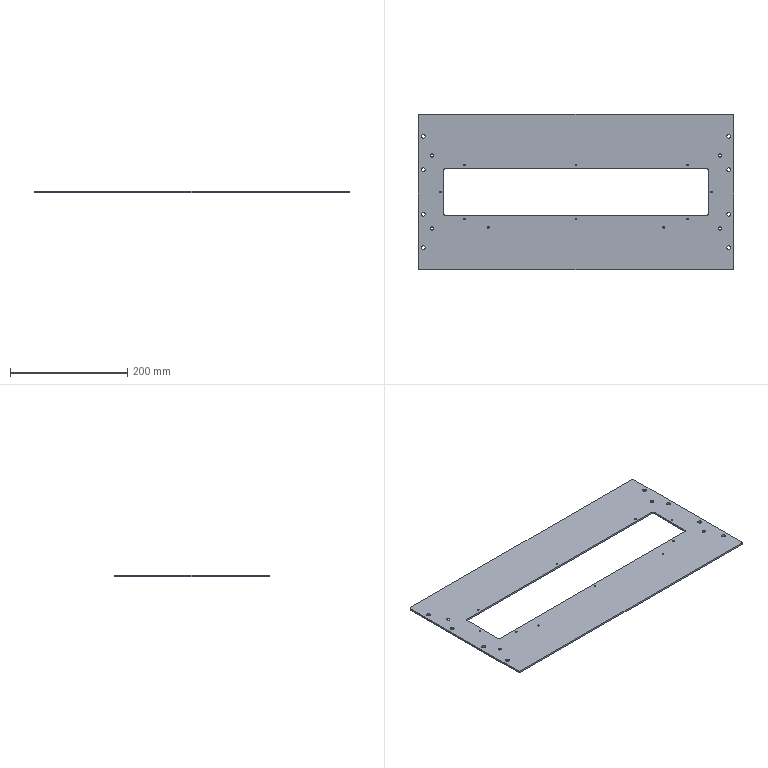CAM job | Mastercam | mm | 6 operations | part box 540 x 266 x 3
1. Contour (Ramp) | 9 - 10 平铣刀
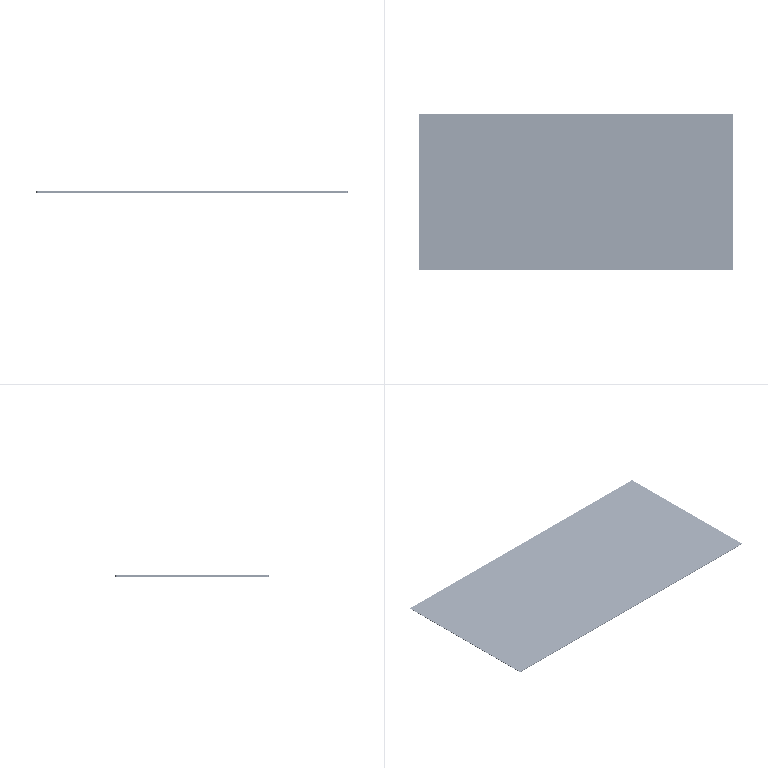2. Contour (2D) | 10 - 10 平铣刀
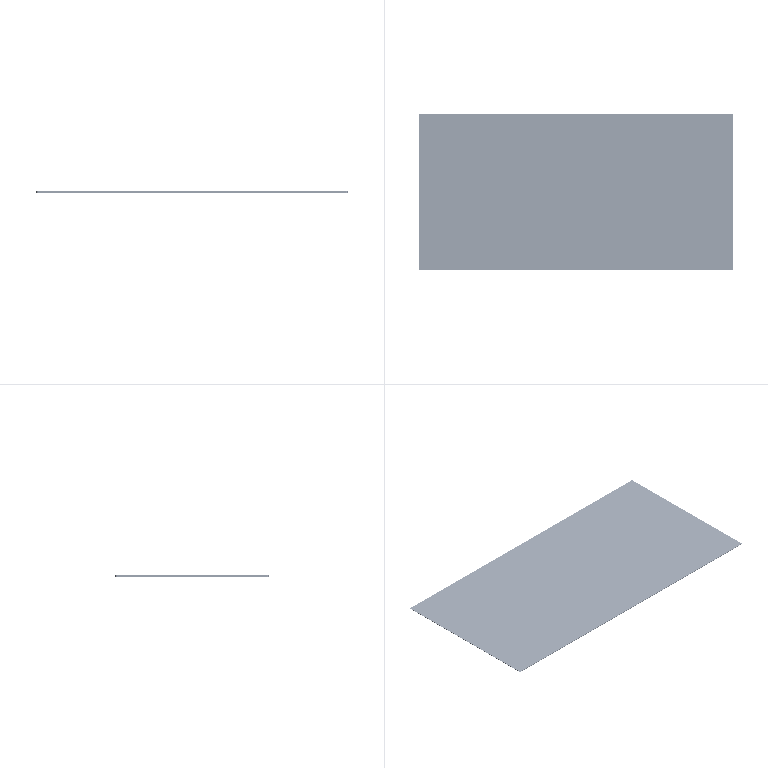3. Contour (Ramp) | 4 - 4 平铣刀
4. Drill/Counterbore | 7 - 4 倒角刀
5. Contour (2D chamfer) | 7 - 4 倒角刀
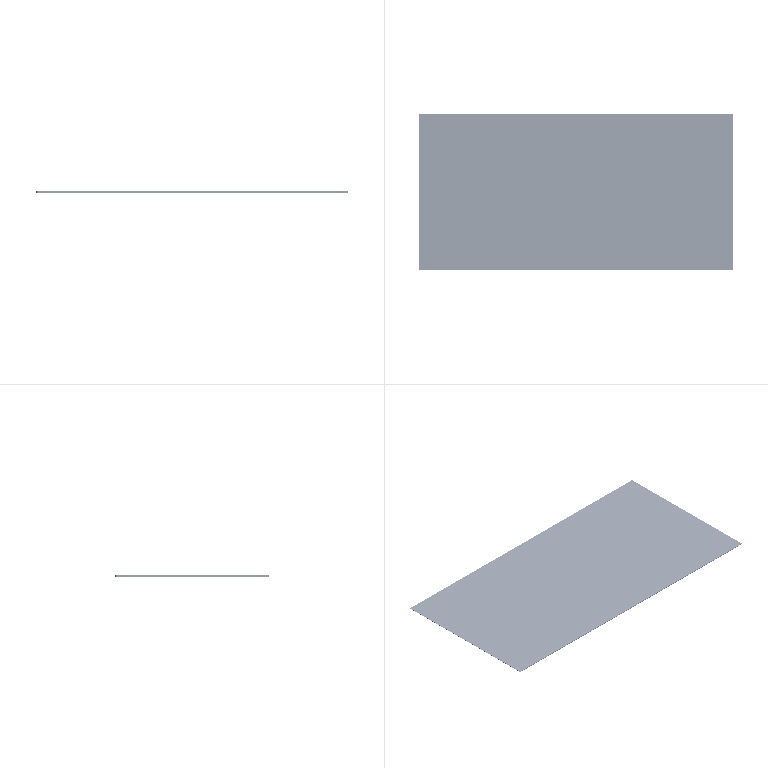6. Contour (2D) | 3 - 3 平铣刀